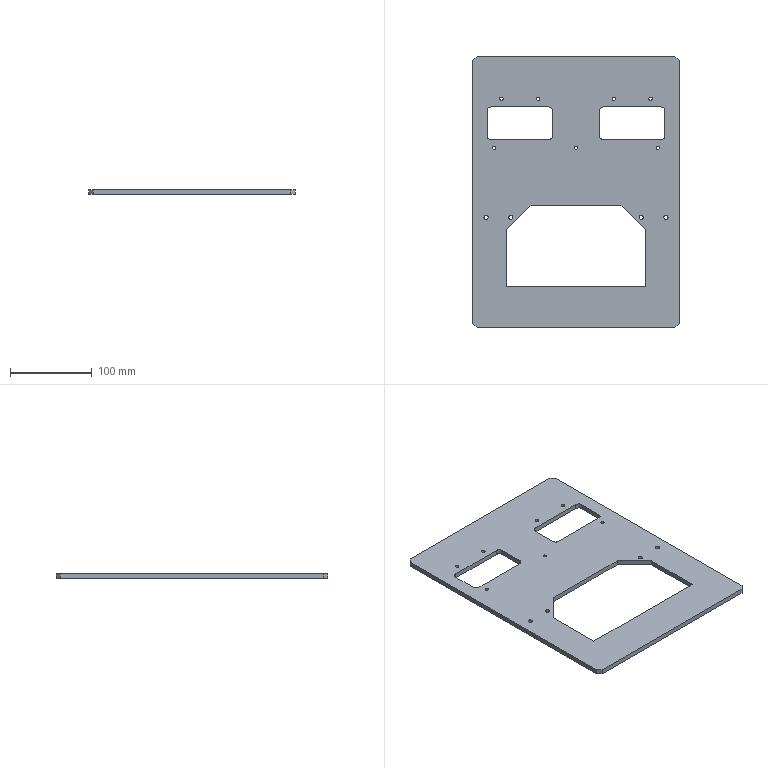Component | SolidWorks | THK-B1009MiddleSpacer-2 | 1 solid | 54 faces | box 252 x 332 x 6 mm | volume 365888 mm3 | cylinder 30 | plane 24 | commonest cylinder face diameters 4.2 x14 5 x8 10 x8 | material Q235A
build123d program:
from build123d import *

# Parameters (mm, degrees)
SKETCH1_W           = 252
SKETCH1_H           = 332
BOSS_EXTRUDE1_DEPTH = 3
SKETCH2_W           = 80
SKETCH2_H           = 40
CUT_EXTRUDE1_DEPTH  = 209.49
FILLET1_R           = 5
CHAMFER1_SIZE       = 5
M6_TAPPED_HOLE1_D   = 5
M5_TAPPED_HOLE1_D   = 4.2


with BuildPart() as part:
    # Sketch1 → Boss-Extrude1 (new, symmetric)
    with BuildSketch(Plane.XY):
        Rectangle(SKETCH1_W, SKETCH1_H)
    extrude(amount=BOSS_EXTRUDE1_DEPTH, both=True)

    # Sketch2 → Cut-Extrude1 (cut, through all)
    with BuildSketch(Plane.XY.offset(3)):
        with Locations((-68.75, 84)):
            Rectangle(SKETCH2_W, SKETCH2_H)
        Polygon((-55, -16), (-85, -46), (-85, -116), (85, -116), (85, -46), (55, -16), align=None)
        with Locations((68.75, 84)):
            Rectangle(SKETCH2_W, SKETCH2_H)
    extrude(amount=-CUT_EXTRUDE1_DEPTH, mode=Mode.SUBTRACT)

    # Fillet1
    fillet1_edges = [part.edges().sort_by_distance(p)[0] for p in [
        (-28.75, 104, 0),
        (-28.75, 64, 0),
        (-108.75, 64, 0),
        (-108.75, 104, 0),
        (108.75, 64, 0),
        (28.75, 64, 0),
        (28.75, 104, 0),
        (108.75, 104, 0),
    ]]
    fillet(fillet1_edges, radius=FILLET1_R)

    # Chamfer1
    chamfer1_edges = [part.edges().sort_by_distance(p)[0] for p in [
        (126, -166, 0),
        (-126, -166, 0),
        (-126, 166, 0),
        (126, 166, 0),
    ]]
    chamfer(chamfer1_edges, length=CHAMFER1_SIZE)

    # M6 Tapped Hole1 (through all)
    with Locations(Plane.XY.offset(3)):
        with Locations((-110, -31), (-80, -31), (80, -31), (110, -31)):
            Hole(M6_TAPPED_HOLE1_D / 2)

    # M5 Tapped Hole1 (through all)
    with Locations(Plane.XY.offset(3)):
        with Locations((-100, 54), (100, 54), (0, 54), (-91.25, 114), (-46.25, 114), (46.25, 114), (91.25, 114)):
            Hole(M5_TAPPED_HOLE1_D / 2)


solid = part.part

# Placed as in the assembly
solid = solid.moved(Location((0, 36, -192), (0, 0, 0)))